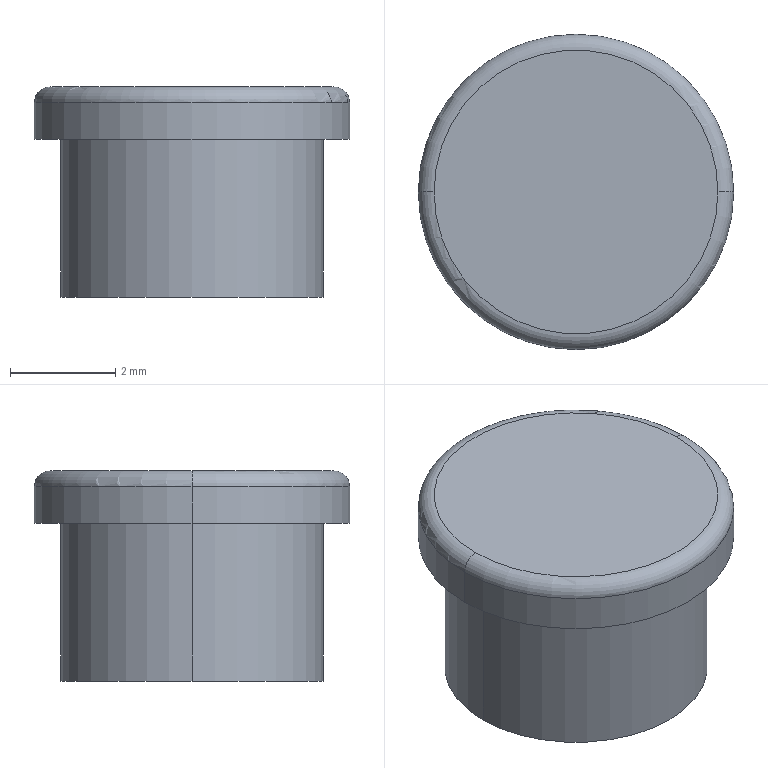Component | SolidWorks | Pin-2 | 1 solid | 9 faces | box 6 x 6 x 4 mm | volume 87 mm3 | cylinder 4 | plane 3 | torus 2 | commonest cylinder face diameters 6 x2 5 x2
build123d program:
from build123d import *

# Parameters (mm, degrees)
SKETCH1_R           = 2.5
BOSS_EXTRUDE1_DEPTH = 3
SKETCH2_R           = 3
BOSS_EXTRUDE2_DEPTH = 1
FILLET1_R           = 0.3


with BuildPart() as part:
    # Sketch1 → Boss-Extrude1 (new body)
    with BuildSketch(Plane.XY):
        Circle(SKETCH1_R)
    extrude(amount=BOSS_EXTRUDE1_DEPTH)

    # Sketch2 → Boss-Extrude2 (add)
    with BuildSketch(Plane.XY.offset(3)):
        Circle(SKETCH2_R)
    extrude(amount=BOSS_EXTRUDE2_DEPTH)

    # Fillet1
    fillet1_edges = [part.edges().sort_by_distance(p)[0] for p in [
        (-3, 0, 4),
    ]]
    fillet(fillet1_edges, radius=FILLET1_R)


solid = part.part

# Placed as in the assembly
solid = solid.moved(Location((-191.5, 220, -140.5), (0, 0, 0)))
STEP:
#1=COLOUR_RGB('',0.7922,0.8196,0.9333);
#2=FILL_AREA_STYLE_COLOUR('',#1);
#3=FILL_AREA_STYLE('',(#2));
#4=SURFACE_STYLE_FILL_AREA(#3);
#5=SURFACE_SIDE_STYLE('',(#4));
#6=SURFACE_STYLE_USAGE(.BOTH.,#5);
#7=PRESENTATION_STYLE_ASSIGNMENT((#6));
#8=CARTESIAN_POINT('',(-7.657,8.661,-5.386));
#9=VERTEX_POINT('',#8);
#10=CARTESIAN_POINT('',(-7.421,8.661,-5.386));
#11=VERTEX_POINT('',#10);
#12=CARTESIAN_POINT('',(-7.539,8.661,-5.386));
#13=DIRECTION('',(0.,0.,-1.));
#14=DIRECTION('',(1.,0.,0.));
#15=AXIS2_PLACEMENT_3D('',#12,#13,#14);
#16=CIRCLE('',#15,0.1181);
#17=EDGE_CURVE('',#9,#11,#16,.T.);
#18=ORIENTED_EDGE('',*,*,#17,.F.);
#19=CARTESIAN_POINT('',(-7.646,8.661,-5.374));
#20=VERTEX_POINT('',#19);
#21=CARTESIAN_POINT('',(-7.646,8.661,-5.386));
#22=DIRECTION('',(0.,1.,0.));
#23=DIRECTION('',(-1.,0.,0.));
#24=AXIS2_PLACEMENT_3D('',#21,#22,#23);
#25=CIRCLE('',#24,0.01181);
#26=EDGE_CURVE('',#9,#20,#25,.T.);
#27=ORIENTED_EDGE('',*,*,#26,.T.);
#28=CARTESIAN_POINT('',(-7.433,8.661,-5.374));
#29=VERTEX_POINT('',#28);
#30=CARTESIAN_POINT('',(-7.539,8.661,-5.374));
#31=DIRECTION('',(0.,0.,1.));
#32=DIRECTION('',(1.,0.,0.));
#33=AXIS2_PLACEMENT_3D('',#30,#31,#32);
#34=CIRCLE('',#33,0.1063);
#35=EDGE_CURVE('',#29,#20,#34,.T.);
#36=ORIENTED_EDGE('',*,*,#35,.F.);
#37=CARTESIAN_POINT('',(-7.433,8.661,-5.386));
#38=DIRECTION('',(0.,-1.,0.));
#39=DIRECTION('',(0.,0.,-1.));
#40=AXIS2_PLACEMENT_3D('',#37,#38,#39);
#41=CIRCLE('',#40,0.01181);
#42=EDGE_CURVE('',#11,#29,#41,.T.);
#43=ORIENTED_EDGE('',*,*,#42,.F.);
#44=EDGE_LOOP('',(#18,#27,#36,#43));
#45=FACE_OUTER_BOUND('',#44,.T.);
#46=CARTESIAN_POINT('',(-7.539,8.661,-5.386));
#47=DIRECTION('',(0.,0.,1.));
#48=DIRECTION('',(1.,0.,0.));
#49=AXIS2_PLACEMENT_3D('',#46,#47,#48);
#50=TOROIDAL_SURFACE('',#49,0.1063,0.01181);
#51=ADVANCED_FACE('',(#45),#50,.T.);
#52=ORIENTED_EDGE('',*,*,#17,.T.);
#53=CARTESIAN_POINT('',(-7.421,8.661,-5.413));
#54=VERTEX_POINT('',#53);
#55=CARTESIAN_POINT('',(-7.421,8.661,-5.374));
#56=DIRECTION('',(0.,0.,-1.));
#57=VECTOR('',#56,39.37);
#58=LINE('',#55,#57);
#59=EDGE_CURVE('',#11,#54,#58,.T.);
#60=ORIENTED_EDGE('',*,*,#59,.T.);
#61=CARTESIAN_POINT('',(-7.657,8.661,-5.413));
#62=VERTEX_POINT('',#61);
#63=CARTESIAN_POINT('',(-7.539,8.661,-5.413));
#64=DIRECTION('',(0.,0.,1.));
#65=DIRECTION('',(1.,0.,0.));
#66=AXIS2_PLACEMENT_3D('',#63,#64,#65);
#67=CIRCLE('',#66,0.1181);
#68=EDGE_CURVE('',#54,#62,#67,.T.);
#69=ORIENTED_EDGE('',*,*,#68,.T.);
#70=CARTESIAN_POINT('',(-7.657,8.661,-5.374));
#71=DIRECTION('',(0.,0.,-1.));
#72=VECTOR('',#71,39.37);
#73=LINE('',#70,#72);
#74=EDGE_CURVE('',#9,#62,#73,.T.);
#75=ORIENTED_EDGE('',*,*,#74,.F.);
#76=EDGE_LOOP('',(#52,#60,#69,#75));
#77=FACE_OUTER_BOUND('',#76,.T.);
#78=CARTESIAN_POINT('',(-7.539,8.661,-5.374));
#79=DIRECTION('',(0.,0.,-1.));
#80=DIRECTION('',(-1.,0.,0.));
#81=AXIS2_PLACEMENT_3D('',#78,#79,#80);
#82=CYLINDRICAL_SURFACE('',#81,0.1181);
#83=ADVANCED_FACE('',(#77),#82,.T.);
#84=CARTESIAN_POINT('',(-7.441,8.661,-5.413));
#85=VERTEX_POINT('',#84);
#86=CARTESIAN_POINT('',(-7.638,8.661,-5.413));
#87=VERTEX_POINT('',#86);
#88=CARTESIAN_POINT('',(-7.539,8.661,-5.413));
#89=DIRECTION('',(0.,0.,1.));
#90=DIRECTION('',(1.,0.,0.));
#91=AXIS2_PLACEMENT_3D('',#88,#89,#90);
#92=CIRCLE('',#91,0.09843);
#93=EDGE_CURVE('',#85,#87,#92,.T.);
#94=ORIENTED_EDGE('',*,*,#93,.F.);
#95=CARTESIAN_POINT('',(-7.441,8.661,-5.531));
#96=VERTEX_POINT('',#95);
#97=CARTESIAN_POINT('',(-7.441,8.661,-5.413));
#98=DIRECTION('',(0.,0.,-1.));
#99=VECTOR('',#98,39.37);
#100=LINE('',#97,#99);
#101=EDGE_CURVE('',#85,#96,#100,.T.);
#102=ORIENTED_EDGE('',*,*,#101,.T.);
#103=CARTESIAN_POINT('',(-7.638,8.661,-5.531));
#104=VERTEX_POINT('',#103);
#105=CARTESIAN_POINT('',(-7.539,8.661,-5.531));
#106=DIRECTION('',(0.,0.,1.));
#107=DIRECTION('',(1.,0.,0.));
#108=AXIS2_PLACEMENT_3D('',#105,#106,#107);
#109=CIRCLE('',#108,0.09843);
#110=EDGE_CURVE('',#96,#104,#109,.T.);
#111=ORIENTED_EDGE('',*,*,#110,.T.);
#112=CARTESIAN_POINT('',(-7.638,8.661,-5.413));
#113=DIRECTION('',(0.,0.,-1.));
#114=VECTOR('',#113,39.37);
#115=LINE('',#112,#114);
#116=EDGE_CURVE('',#87,#104,#115,.T.);
#117=ORIENTED_EDGE('',*,*,#116,.F.);
#118=EDGE_LOOP('',(#94,#102,#111,#117));
#119=FACE_OUTER_BOUND('',#118,.T.);
#120=CARTESIAN_POINT('',(-7.539,8.661,-5.413));
#121=DIRECTION('',(0.,0.,-1.));
#122=DIRECTION('',(-1.,0.,0.));
#123=AXIS2_PLACEMENT_3D('',#120,#121,#122);
#124=CYLINDRICAL_SURFACE('',#123,0.09843);
#125=ADVANCED_FACE('',(#119),#124,.T.);
#126=ORIENTED_EDGE('',*,*,#101,.F.);
#127=CARTESIAN_POINT('',(-7.539,8.661,-5.413));
#128=DIRECTION('',(0.,0.,1.));
#129=DIRECTION('',(1.,0.,0.));
#130=AXIS2_PLACEMENT_3D('',#127,#128,#129);
#131=CIRCLE('',#130,0.09843);
#132=EDGE_CURVE('',#87,#85,#131,.T.);
#133=ORIENTED_EDGE('',*,*,#132,.F.);
#134=ORIENTED_EDGE('',*,*,#116,.T.);
#135=CARTESIAN_POINT('',(-7.539,8.661,-5.531));
#136=DIRECTION('',(0.,0.,1.));
#137=DIRECTION('',(1.,0.,0.));
#138=AXIS2_PLACEMENT_3D('',#135,#136,#137);
#139=CIRCLE('',#138,0.09843);
#140=EDGE_CURVE('',#104,#96,#139,.T.);
#141=ORIENTED_EDGE('',*,*,#140,.T.);
#142=EDGE_LOOP('',(#126,#133,#134,#141));
#143=FACE_OUTER_BOUND('',#142,.T.);
#144=CARTESIAN_POINT('',(-7.539,8.661,-5.413));
#145=DIRECTION('',(0.,0.,-1.));
#146=DIRECTION('',(-1.,0.,0.));
#147=AXIS2_PLACEMENT_3D('',#144,#145,#146);
#148=CYLINDRICAL_SURFACE('',#147,0.09843);
#149=ADVANCED_FACE('',(#143),#148,.T.);
#150=ORIENTED_EDGE('',*,*,#140,.F.);
#151=ORIENTED_EDGE('',*,*,#110,.F.);
#152=EDGE_LOOP('',(#150,#151));
#153=FACE_OUTER_BOUND('',#152,.T.);
#154=CARTESIAN_POINT('',(-7.539,8.661,-5.531));
#155=DIRECTION('',(0.,0.,1.));
#156=DIRECTION('',(1.,0.,0.));
#157=AXIS2_PLACEMENT_3D('',#154,#155,#156);
#158=PLANE('',#157);
#159=ADVANCED_FACE('',(#153),#158,.F.);
#160=ORIENTED_EDGE('',*,*,#59,.F.);
#161=CARTESIAN_POINT('',(-7.539,8.661,-5.386));
#162=DIRECTION('',(0.,0.,-1.));
#163=DIRECTION('',(1.,0.,0.));
#164=AXIS2_PLACEMENT_3D('',#161,#162,#163);
#165=CIRCLE('',#164,0.1181);
#166=EDGE_CURVE('',#11,#9,#165,.T.);
#167=ORIENTED_EDGE('',*,*,#166,.T.);
#168=ORIENTED_EDGE('',*,*,#74,.T.);
#169=CARTESIAN_POINT('',(-7.539,8.661,-5.413));
#170=DIRECTION('',(0.,0.,1.));
#171=DIRECTION('',(1.,0.,0.));
#172=AXIS2_PLACEMENT_3D('',#169,#170,#171);
#173=CIRCLE('',#172,0.1181);
#174=EDGE_CURVE('',#62,#54,#173,.T.);
#175=ORIENTED_EDGE('',*,*,#174,.T.);
#176=EDGE_LOOP('',(#160,#167,#168,#175));
#177=FACE_OUTER_BOUND('',#176,.T.);
#178=CARTESIAN_POINT('',(-7.539,8.661,-5.374));
#179=DIRECTION('',(0.,0.,-1.));
#180=DIRECTION('',(-1.,0.,0.));
#181=AXIS2_PLACEMENT_3D('',#178,#179,#180);
#182=CYLINDRICAL_SURFACE('',#181,0.1181);
#183=ADVANCED_FACE('',(#177),#182,.T.);
#184=ORIENTED_EDGE('',*,*,#35,.T.);
#185=CARTESIAN_POINT('',(-7.539,8.661,-5.374));
#186=DIRECTION('',(0.,0.,1.));
#187=DIRECTION('',(1.,0.,0.));
#188=AXIS2_PLACEMENT_3D('',#185,#186,#187);
#189=CIRCLE('',#188,0.1063);
#190=EDGE_CURVE('',#20,#29,#189,.T.);
#191=ORIENTED_EDGE('',*,*,#190,.T.);
#192=EDGE_LOOP('',(#184,#191));
#193=FACE_OUTER_BOUND('',#192,.T.);
#194=CARTESIAN_POINT('',(-7.539,8.661,-5.374));
#195=DIRECTION('',(0.,0.,1.));
#196=DIRECTION('',(1.,0.,0.));
#197=AXIS2_PLACEMENT_3D('',#194,#195,#196);
#198=PLANE('',#197);
#199=ADVANCED_FACE('',(#193),#198,.T.);
#200=ORIENTED_EDGE('',*,*,#132,.T.);
#201=ORIENTED_EDGE('',*,*,#93,.T.);
#202=EDGE_LOOP('',(#200,#201));
#203=FACE_BOUND('',#202,.T.);
#204=ORIENTED_EDGE('',*,*,#174,.F.);
#205=ORIENTED_EDGE('',*,*,#68,.F.);
#206=EDGE_LOOP('',(#204,#205));
#207=FACE_OUTER_BOUND('',#206,.T.);
#208=CARTESIAN_POINT('',(-7.539,8.661,-5.413));
#209=DIRECTION('',(0.,0.,1.));
#210=DIRECTION('',(1.,0.,0.));
#211=AXIS2_PLACEMENT_3D('',#208,#209,#210);
#212=PLANE('',#211);
#213=ADVANCED_FACE('',(#203,#207),#212,.F.);
#214=ORIENTED_EDGE('',*,*,#26,.F.);
#215=ORIENTED_EDGE('',*,*,#166,.F.);
#216=ORIENTED_EDGE('',*,*,#42,.T.);
#217=ORIENTED_EDGE('',*,*,#190,.F.);
#218=EDGE_LOOP('',(#214,#215,#216,#217));
#219=FACE_OUTER_BOUND('',#218,.T.);
#220=CARTESIAN_POINT('',(-7.539,8.661,-5.386));
#221=DIRECTION('',(0.,0.,1.));
#222=DIRECTION('',(1.,0.,0.));
#223=AXIS2_PLACEMENT_3D('',#220,#221,#222);
#224=TOROIDAL_SURFACE('',#223,0.1063,0.01181);
#225=ADVANCED_FACE('',(#219),#224,.T.);
#226=CLOSED_SHELL('',(#51,#83,#125,#149,#159,#183,#199,#213,#225));
#227=MANIFOLD_SOLID_BREP('',#226);
#228=STYLED_ITEM('',(#7),#227);
#229=PRESENTATION_LAYER_ASSIGNMENT('','',(#228));
#230=(LENGTH_UNIT()NAMED_UNIT(*)SI_UNIT($,.METRE.));
#231=LENGTH_MEASURE_WITH_UNIT(LENGTH_MEASURE(0.0254),#230);
#232=DIMENSIONAL_EXPONENTS(1.,0.,0.,0.,0.,0.,0.);
#233=(CONVERSION_BASED_UNIT('',#231)LENGTH_UNIT()NAMED_UNIT(#232));
#234=UNCERTAINTY_MEASURE_WITH_UNIT(LENGTH_MEASURE(0.00001),#233,'','');
#235=(NAMED_UNIT(*)PLANE_ANGLE_UNIT()SI_UNIT($,.RADIAN.));
#236=(NAMED_UNIT(*)SI_UNIT($,.STERADIAN.)SOLID_ANGLE_UNIT());
#237=(GEOMETRIC_REPRESENTATION_CONTEXT(3)GLOBAL_UNCERTAINTY_ASSIGNED_CONTEXT((#234))GLOBAL_UNIT_ASSIGNED_CONTEXT((#233,#235,#236))REPRESENTATION_CONTEXT('',''));
#238=MECHANICAL_DESIGN_GEOMETRIC_PRESENTATION_REPRESENTATION('',(#228),#237);
#239=CARTESIAN_POINT('',(0.,0.,0.));
#240=DIRECTION('',(0.,0.,1.));
#241=DIRECTION('',(1.,0.,0.));
#242=AXIS2_PLACEMENT_3D('',#239,#240,#241);
#243=(LENGTH_UNIT()NAMED_UNIT(*)SI_UNIT($,.METRE.));
#244=LENGTH_MEASURE_WITH_UNIT(LENGTH_MEASURE(0.0254),#243);
#245=DIMENSIONAL_EXPONENTS(1.,0.,0.,0.,0.,0.,0.);
#246=(CONVERSION_BASED_UNIT('',#244)LENGTH_UNIT()NAMED_UNIT(#245));
#247=UNCERTAINTY_MEASURE_WITH_UNIT(LENGTH_MEASURE(0.00001),#246,'','');
#248=(NAMED_UNIT(*)PLANE_ANGLE_UNIT()SI_UNIT($,.RADIAN.));
#249=(NAMED_UNIT(*)SI_UNIT($,.STERADIAN.)SOLID_ANGLE_UNIT());
#250=(GEOMETRIC_REPRESENTATION_CONTEXT(3)GLOBAL_UNCERTAINTY_ASSIGNED_CONTEXT((#247))GLOBAL_UNIT_ASSIGNED_CONTEXT((#246,#248,#249))REPRESENTATION_CONTEXT('',''));
#251=ADVANCED_BREP_SHAPE_REPRESENTATION('',(#227,#242),#250);